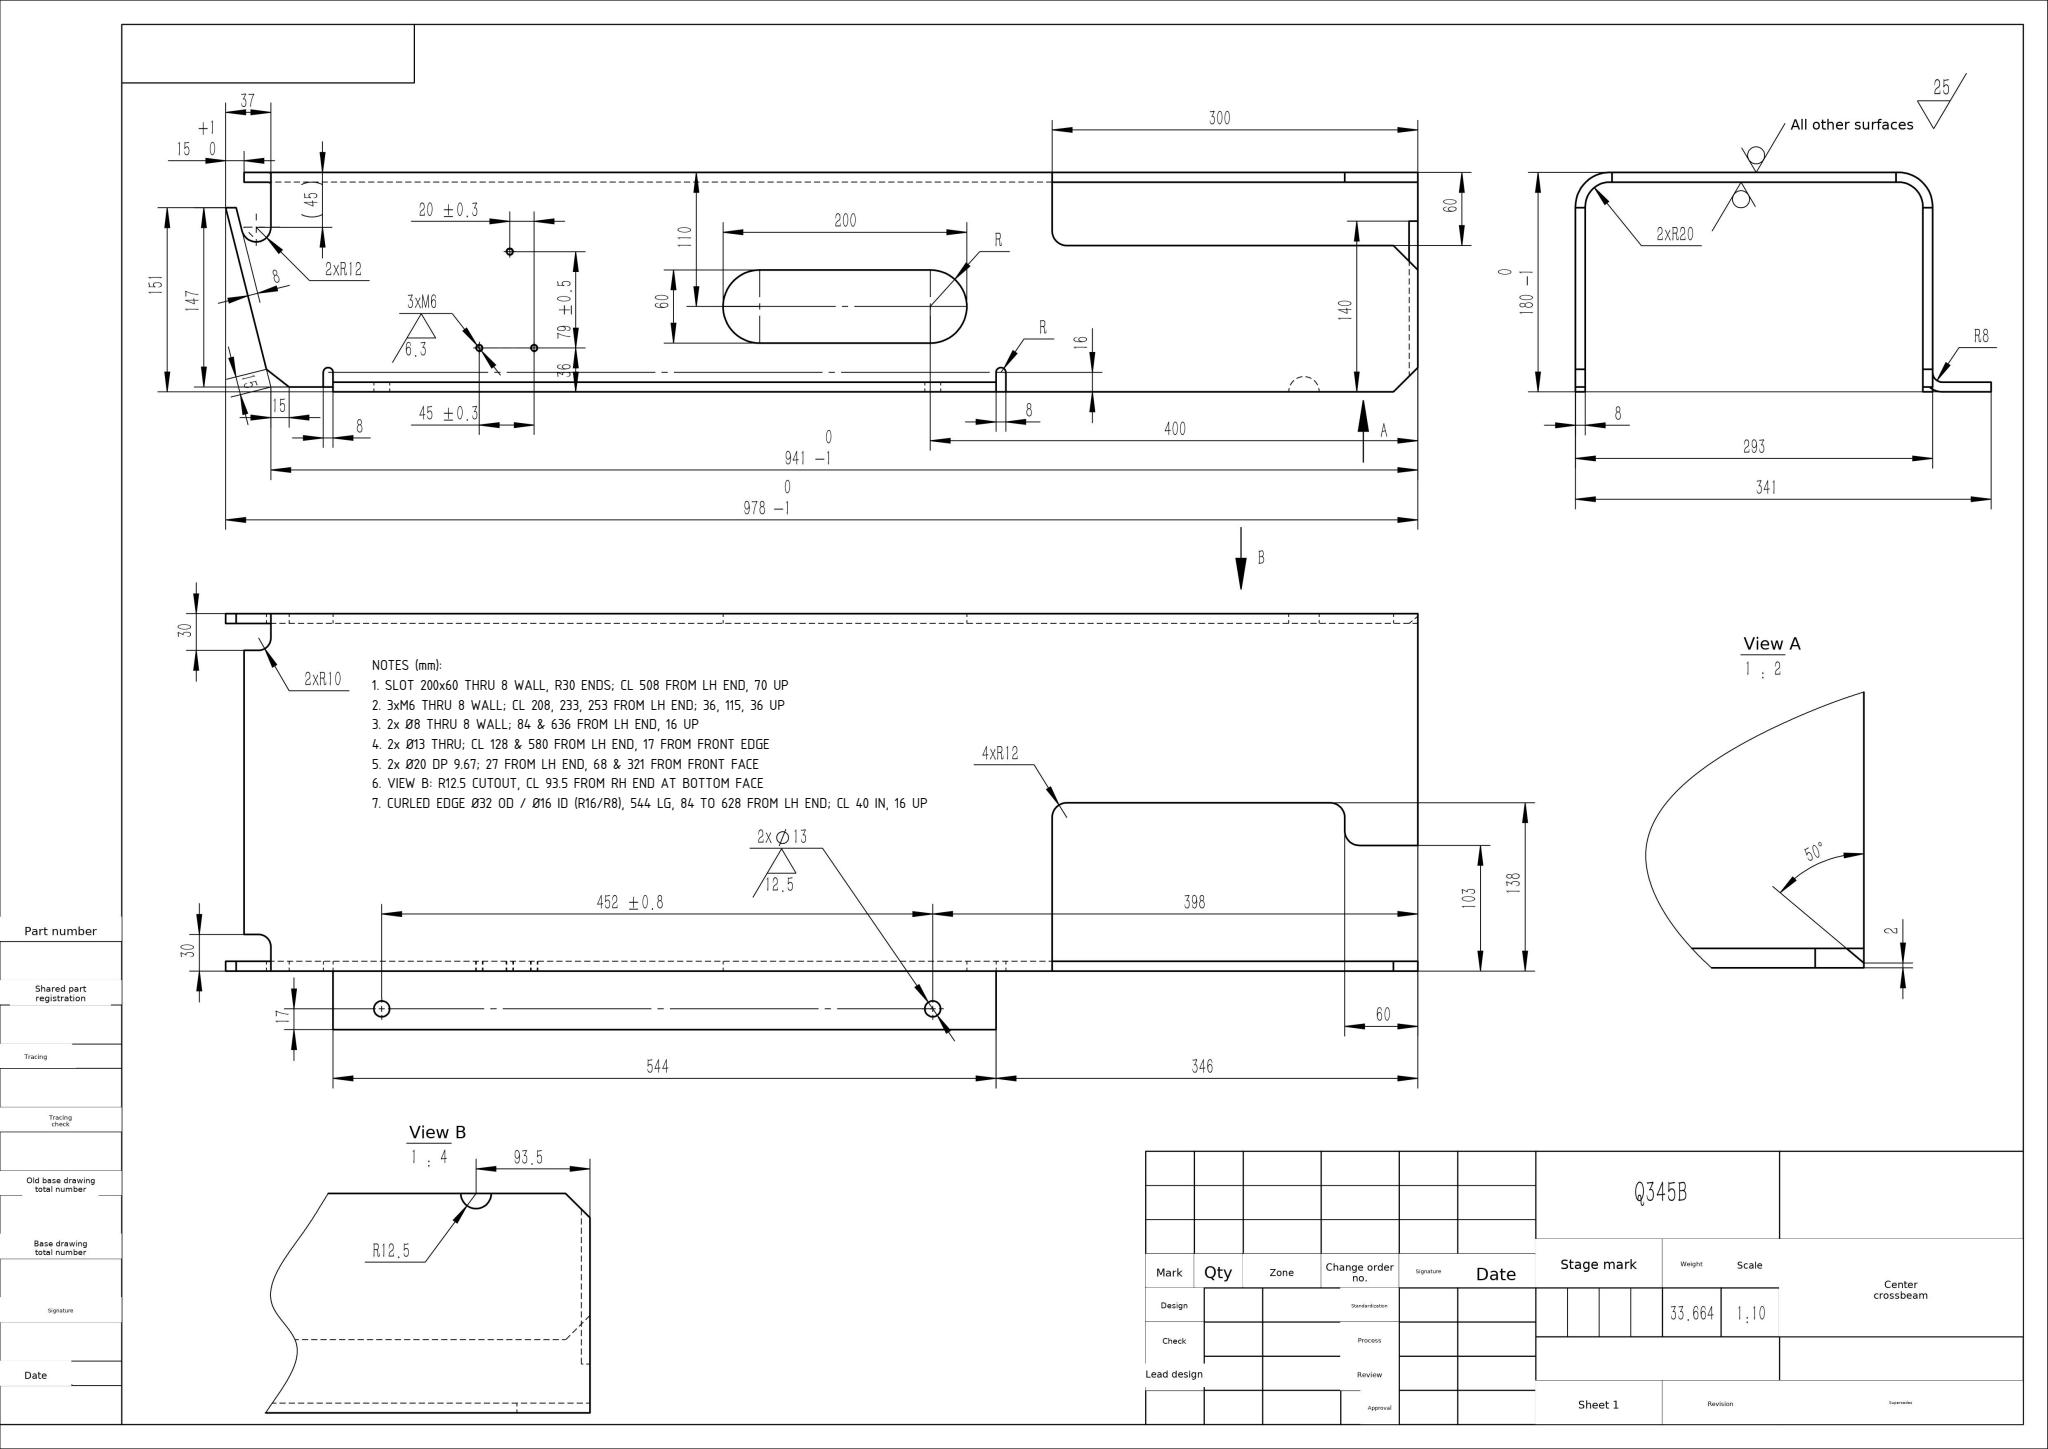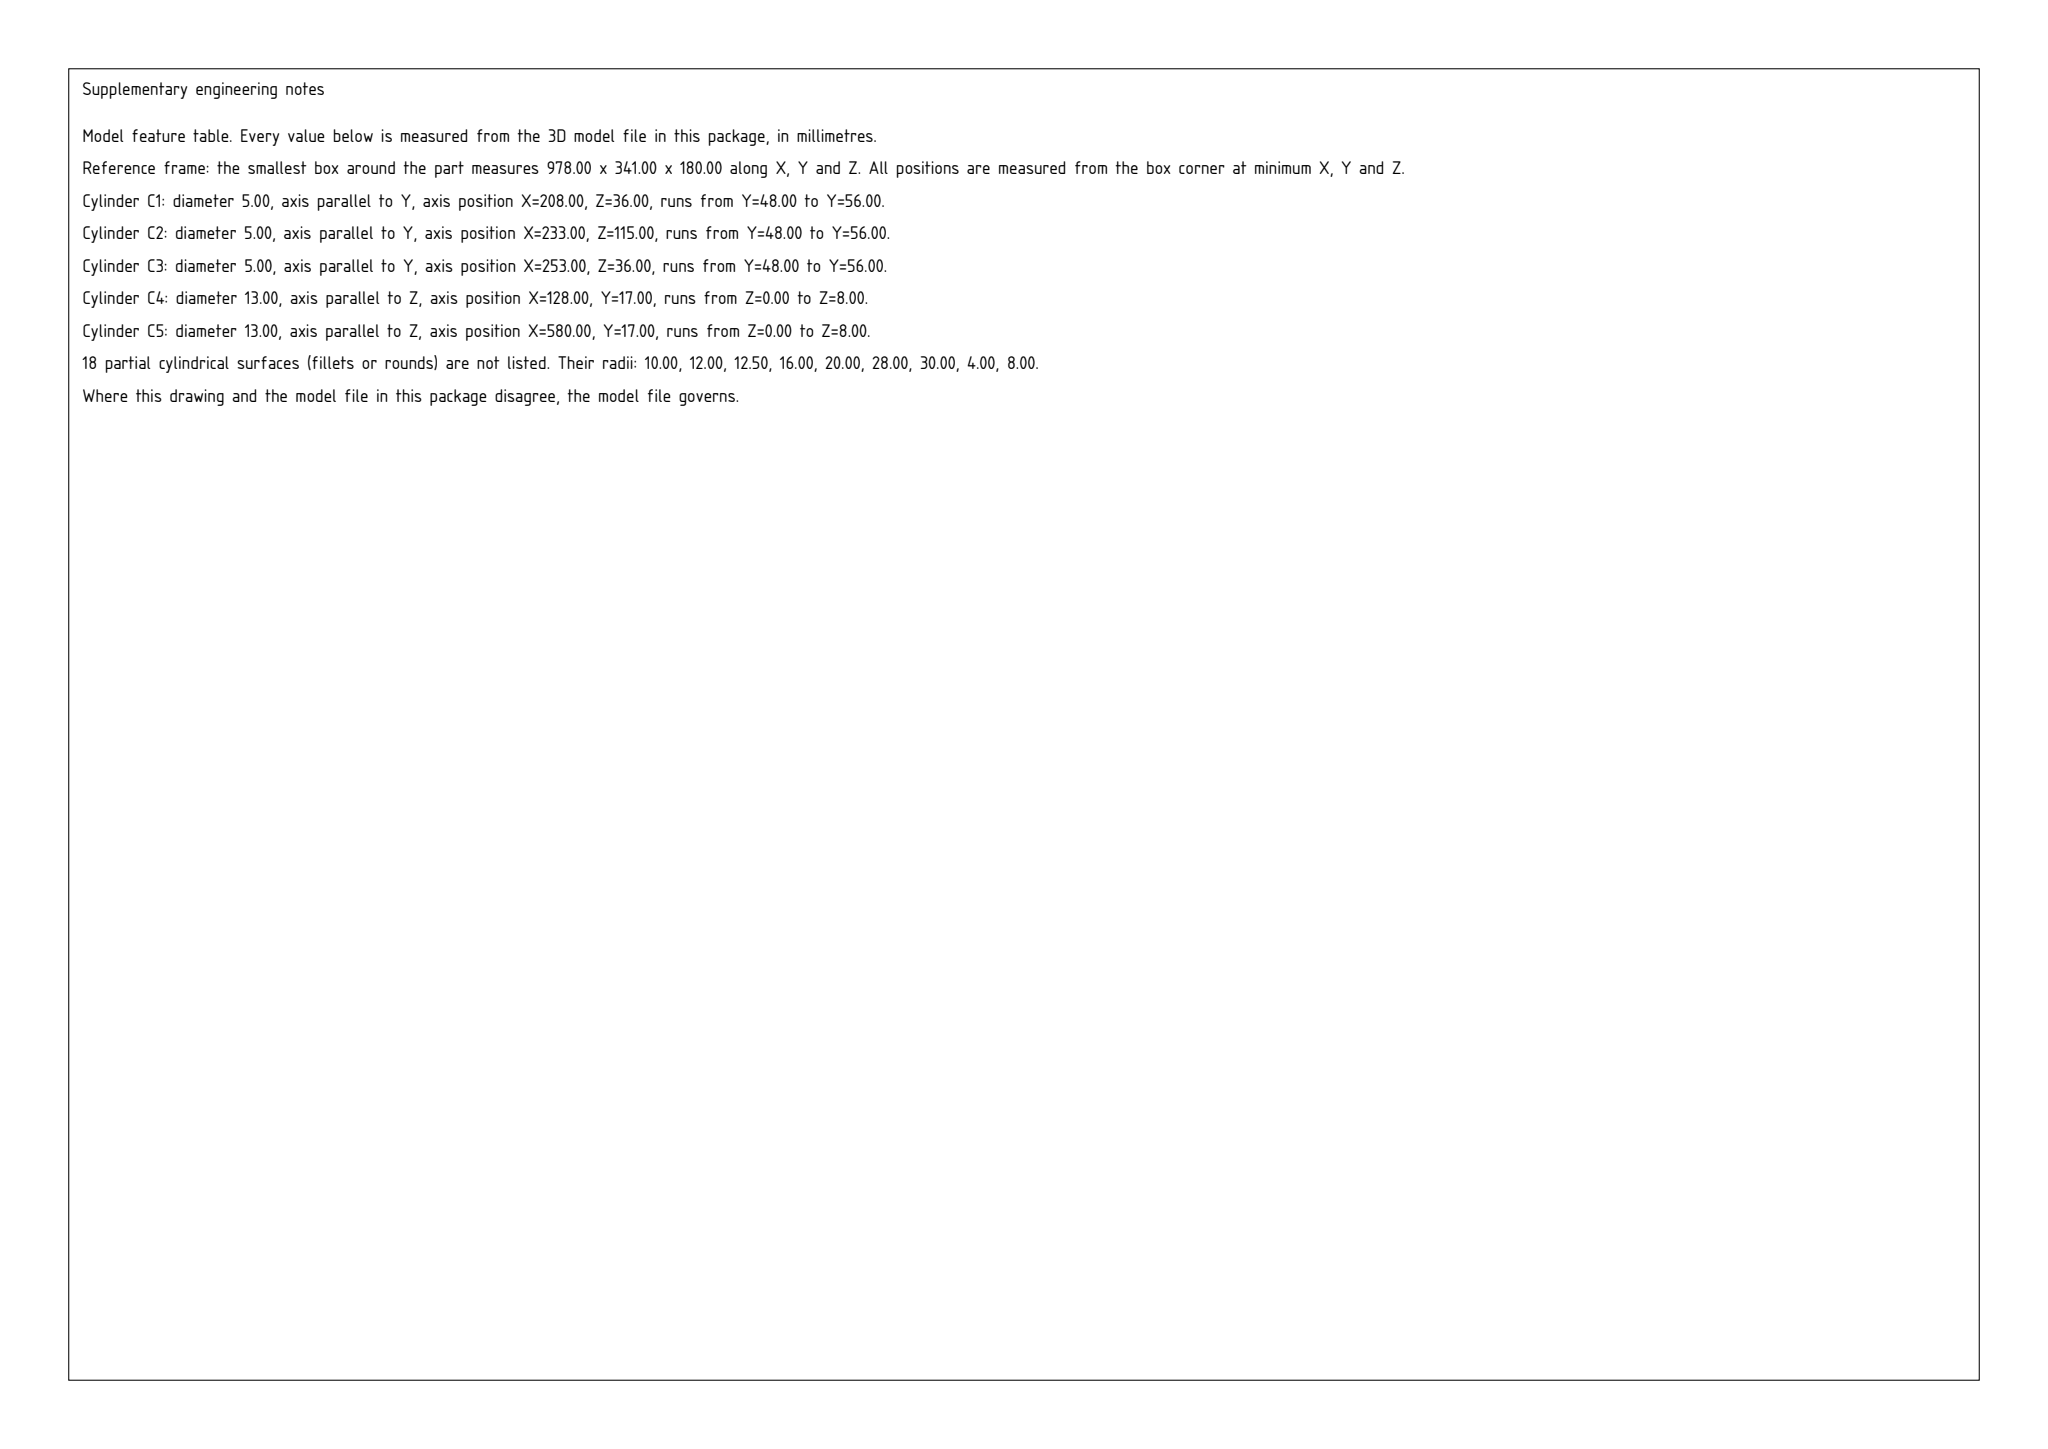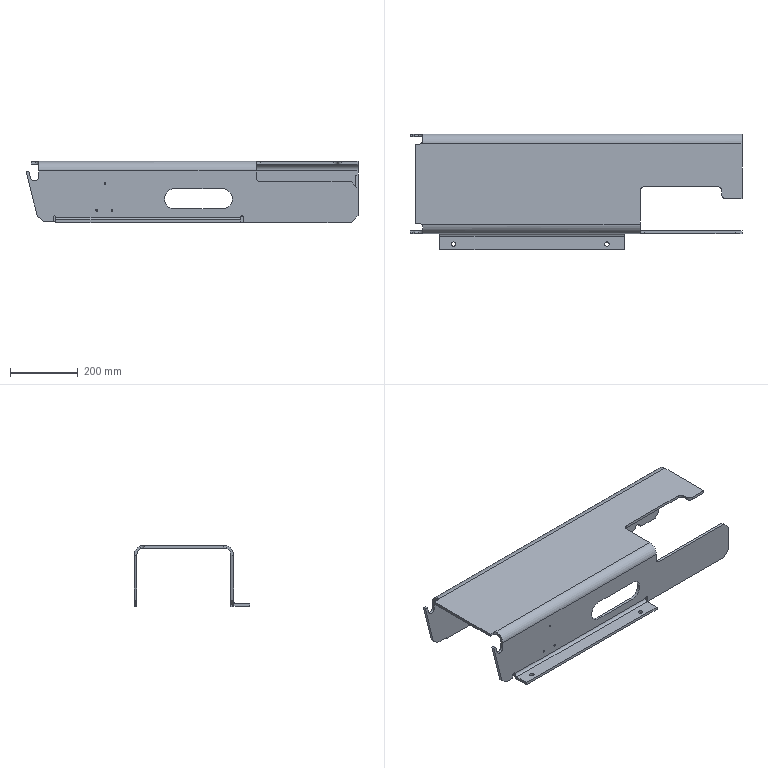Part | SolidWorks | mm | 1 solid | 81 faces | box 978 x 341 x 180 mm | volume 4288401 mm3 | plane 48 | cylinder 33 | commonest cylinder face diameters 24 x8 5 x6 13 x4 60 x4 20 x2 8 x2 40 x2 56 x2
Drawing notes:
SLOT 200x60 THRU 8 WALL, R30 ENDS; CL 508 FROM LH END, 70 UP | from the solid: 2x Ø60 y-axis cyls len 8 at x=438 & 578, z=70 -> R30 ends, 140 CL spacing, 200 overall, CL x=508
3xM6 THRU 8 WALL; CL 208, 233, 253 FROM LH END; 36, 115, 36 UP | from the solid: Ø5 y-axis cyls len 8 at (208,36),(233,115),(253,36); wall 8 thk between x planes 80/88
2x Ø8 THRU 8 WALL; 84 & 636 FROM LH END, 16 UP | from the solid: Ø8 y-axis cyls len 8 at [84,-,16] and [636,-,16]
2x Ø13 THRU; CL 128 & 580 FROM LH END, 17 FROM FRONT EDGE | from the solid: Ø13 z-axis cyls len 8 at [128,17] and [580,17]; 580-128=452 matches sheet
2x Ø20 DP 9.67; 27 FROM LH END, 68 & 321 FROM FRONT FACE | from the solid: Ø20 z-axis cyls len 9.67 at [27,68] and [27,321]
VIEW B: R12.5 CUTOUT, CL 93.5 FROM RH END AT BOTTOM FACE | from the solid: Ø25 y-axis cyl at x=884.5, z=0, len 8; 978-884.5=93.5 from RH end
CURLED EDGE Ø32 OD / Ø16 ID (R16/R8), 544 LG, 84 TO 628 FROM LH END; CL 40 IN, 16 UP | from the solid: Ø32 and Ø16 x-axis cyls, len 544, at y=40, z=16; start x=84 -> 84+544=628
build123d program:
from build123d import *

# Parameters (mm, degrees)
BOSS_EXTRUDE1_DEPTH   = 8
SKETCH2_W             = 978
SKETCH2_H             = 8
BOSS_EXTRUDE2_DEPTH   = 172
SKETCH3_OUTSIDE_W     = 1187.338
SKETCH3_OUTSIDE_H     = 389.338
CUT_EXTRUDE1_DEPTH    = 8
SKETCH4_OUTSIDE_W     = 1187.338
SKETCH4_OUTSIDE_H     = 389.338
CUT_EXTRUDE2_DEPTH    = 8
CUT_EXTRUDE3_DEPTH    = 140
M6_TAPPED_HOLE1_D     = 5
M6_TAPPED_HOLE1_DEPTH = 8
SKETCH8_W             = 544
SKETCH8_H             = 8
BOSS_EXTRUDE3_DEPTH   = 48
SKETCH9_R             = 6.5
CUT_EXTRUDE4_DEPTH    = 1001.457
FILLET1_R             = 8
FILLET2_R             = 16
FILLET3_R             = 20
FILLET4_R             = 28


with BuildPart() as part:
    # Sketch1 → Boss-Extrude1 (new body)
    with BuildSketch(Plane.XY):
        with BuildLine():
            Line((-22, 263), (-10, 263))
            ThreePointArc((-10, 263), (-2.929, 265.929), (0, 273))
            Line((0, 273), (0, 293))
            Line((0, 293), (941, 293))
            Line((941, 293), (941, 103))
            Line((941, 103), (893, 103))
            ThreePointArc((893, 103), (884.515, 106.515), (881, 115))
            Line((881, 115), (881, 126))
            ThreePointArc((881, 126), (877.485, 134.485), (869, 138))
            Line((869, 138), (653, 138))
            ThreePointArc((653, 138), (644.515, 134.485), (641, 126))
            Line((641, 126), (641, 0))
            Line((641, 0), (0, 0))
            Line((0, 0), (0, 20))
            ThreePointArc((0, 20), (-2.929, 27.071), (-10, 30))
            Line((-10, 30), (-22, 30))
            Line((-22, 30), (-22, 263))
        make_face()
    extrude(amount=BOSS_EXTRUDE1_DEPTH)

    # Sketch2 → Boss-Extrude2 (add)
    with BuildSketch(Plane(origin=(0, 0, 0), x_dir=(-1, 0, 0), z_dir=(0, 0, -1))):
        with Locations((-452, 4)):
            Rectangle(SKETCH2_W, SKETCH2_H)
        with Locations((-452, 289)):
            Rectangle(SKETCH2_W, SKETCH2_H)
    extrude(amount=BOSS_EXTRUDE2_DEPTH)

    # Sketch3 outside → Cut-Extrude1 (cut)
    # profile 1 of 2: a face of its own
    with BuildSketch(Plane(origin=(0, 0, 0), x_dir=(-1, 0, 0), z_dir=(0, -1, 0))):
        with Locations((-452, 82)):
            Rectangle(SKETCH3_OUTSIDE_W, SKETCH3_OUTSIDE_H)
        with BuildLine():
            Line((0, -8), (0, 37))
            ThreePointArc((0, 37), (10.524, 48.909), (23.637, 39.929))
            Line((23.637, 39.929), (28.401, 21))
            Line((28.401, 21), (37, 21))
            Line((37, 21), (3.661, 153.454))
            Line((3.661, 153.454), (-15, 168))
            Line((-15, 168), (-43, 168))
            Line((-43, 168), (-43, 156))
            ThreePointArc((-43, 156), (-47, 152), (-51, 156))
            Line((-51, 156), (-51, 172))
            Line((-51, 172), (-595, 172))
            Line((-595, 172), (-595, 156))
            ThreePointArc((-595, 156), (-599, 152), (-603, 156))
            Line((-603, 156), (-603, 172))
            Line((-603, 172), (-921, 172))
            Line((-921, 172), (-941, 152))
            Line((-941, 152), (-941, 72))
            Line((-941, 72), (-921, 52))
            Line((-921, 52), (-653, 52))
            ThreePointArc((-653, 52), (-644.515, 48.485), (-641, 40))
            Line((-641, 40), (-641, -8))
            Line((-641, -8), (0, -8))
        make_face(mode=Mode.SUBTRACT)
    # profile 2 of 2: a face of its own
    with BuildSketch(Plane(origin=(0, 0, 0), x_dir=(-1, 0, 0), z_dir=(0, -1, 0))):
        with BuildLine():
            Line((-401, 72), (-541, 72))
            ThreePointArc((-541, 72), (-571, 102), (-541, 132))
            Line((-541, 132), (-401, 132))
            ThreePointArc((-401, 132), (-371, 102), (-401, 72))
        make_face()
    extrude(amount=-CUT_EXTRUDE1_DEPTH, mode=Mode.SUBTRACT)

    # Sketch4 outside → Cut-Extrude2 (cut)
    # profile 1 of 2: a face of its own
    with BuildSketch(Plane(origin=(0, 285, 0), x_dir=(-1, 0, 0), z_dir=(0, -1, 0))):
        with Locations((-452, 82)):
            Rectangle(SKETCH4_OUTSIDE_W, SKETCH4_OUTSIDE_H)
        with BuildLine():
            Line((0, -8), (0, 37))
            ThreePointArc((0, 37), (10.524, 48.909), (23.637, 39.929))
            Line((23.637, 39.929), (28.401, 21))
            Line((28.401, 21), (37, 21))
            Line((37, 21), (3.661, 153.454))
            Line((3.661, 153.454), (-15, 168))
            Line((-15, 168), (-51, 168))
            Line((-51, 168), (-51, 172))
            Line((-51, 172), (-835, 172))
            ThreePointArc((-835, 172), (-847.5, 159.5), (-860, 172))
            Line((-860, 172), (-921, 172))
            Line((-921, 172), (-941, 152))
            Line((-941, 152), (-941, -8))
            Line((-941, -8), (0, -8))
        make_face(mode=Mode.SUBTRACT)
    # profile 2 of 2: a face of its own
    with BuildSketch(Plane(origin=(0, 285, 0), x_dir=(-1, 0, 0), z_dir=(0, -1, 0))):
        with BuildLine():
            Line((-541, 132), (-401, 132))
            ThreePointArc((-401, 132), (-371, 102), (-401, 72))
            Line((-401, 72), (-541, 72))
            ThreePointArc((-541, 72), (-571, 102), (-541, 132))
        make_face()
    extrude(amount=-CUT_EXTRUDE2_DEPTH, mode=Mode.SUBTRACT)

    # Sketch5 → Cut-Extrude3 (cut)
    with BuildSketch(Plane(origin=(0, 0, -172), x_dir=(-1, 0, 0), z_dir=(0, 0, -1))):
        Polygon((-941, 291), (-933.849, 285), (-941, 285), align=None)
    extrude(amount=-CUT_EXTRUDE3_DEPTH, mode=Mode.SUBTRACT)

    # M6 Tapped Hole1
    with Locations(Plane(origin=(196, 0, -57), x_dir=(0, 0, -1), z_dir=(0, -1, 0))):
        with Locations((0, 0), (79, -25), (79, 20)):
            Hole(M6_TAPPED_HOLE1_D / 2, depth=M6_TAPPED_HOLE1_DEPTH)

    # Sketch8 → Boss-Extrude3 (add)
    with BuildSketch(Plane(origin=(0, 0, 0), x_dir=(-1, 0, 0), z_dir=(0, -1, 0))):
        with Locations((-323, 168)):
            Rectangle(SKETCH8_W, SKETCH8_H)
    extrude(amount=BOSS_EXTRUDE3_DEPTH)

    # Sketch9 → Cut-Extrude4 (cut, through all)
    with BuildSketch(Plane.XY.offset(-164)):
        with Locations((91, -31)):
            Circle(SKETCH9_R)
        with Locations((543, -31)):
            Circle(SKETCH9_R)
    extrude(amount=-CUT_EXTRUDE4_DEPTH, mode=Mode.SUBTRACT)

    # Fillet1
    fillet1_edges = [part.edges().sort_by_distance(p)[0] for p in [
        (323, 0, -164),
    ]]
    fillet(fillet1_edges, radius=FILLET1_R)

    # Fillet2
    fillet2_edges = [part.edges().sort_by_distance(p)[0] for p in [
        (323, 8, -172),
    ]]
    fillet(fillet2_edges, radius=FILLET2_R)

    # Fillet3
    fillet3_edges = [part.edges().sort_by_distance(p)[0] for p in [
        (470.5, 285, 0),
        (320.5, 8, 0),
    ]]
    fillet(fillet3_edges, radius=FILLET3_R)

    # Fillet4
    fillet4_edges = [part.edges().sort_by_distance(p)[0] for p in [
        (470.5, 293, 8),
        (320.5, 0, 8),
    ]]
    fillet(fillet4_edges, radius=FILLET4_R)


solid = part.part